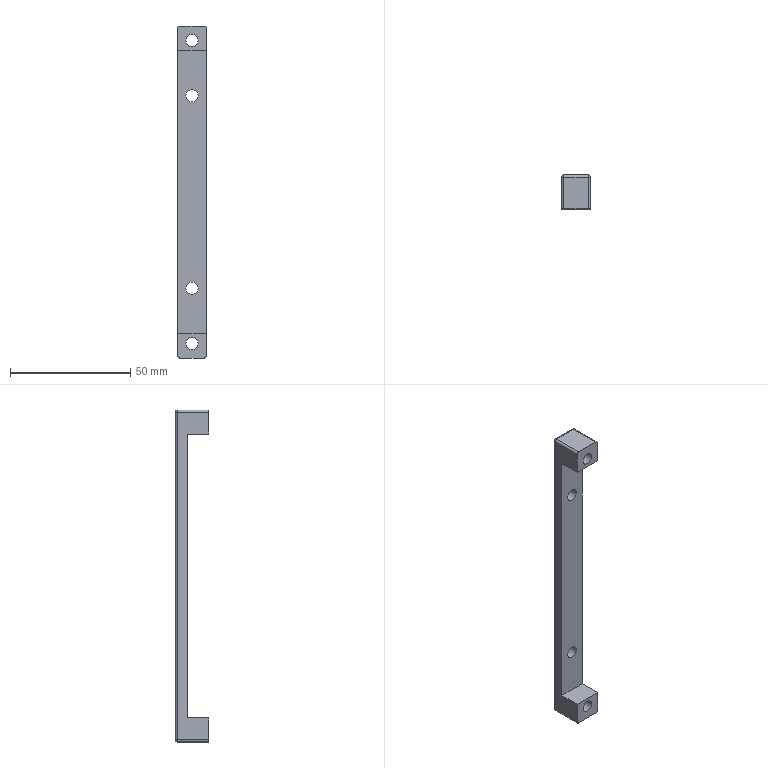Component | SolidWorks | 120.1-1 | 1 solid | 30 faces | box 12 x 14 x 138 mm | volume 9618 mm3 | cylinder 16 | plane 10 | sphere 4 | commonest cylinder face diameters 5 x8 2 x8
build123d program:
from build123d import *

# Parameters (mm, degrees)
SKETCH2_W                    = 138
SKETCH2_H                    = 12
BOSS_EXTRUDE1_DEPTH          = 14
SKETCH3_W                    = 118
SKETCH3_H                    = 9
CUT_EXTRUDE1_DEPTH           = 14
F_5_0_5_DIAMETER_HOLE1_D     = 5
F_5_0_5_DIAMETER_HOLE1_DEPTH = 15
F_5_0_5_DIAMETER_HOLE1_TIP   = 1.502
F_5_0_5_DIAMETER_HOLE2_D     = 5
F_5_0_5_DIAMETER_HOLE2_DEPTH = 10.1
F_5_0_5_DIAMETER_HOLE2_TIP   = 1.502
FILLET1_R                    = 1


with BuildPart() as part:
    # Sketch2 → Boss-Extrude1 (new body)
    with BuildSketch(Plane(origin=(0, 0, 0), x_dir=(1, 0, 0), z_dir=(0, 1, 0))):
        Rectangle(SKETCH2_W, SKETCH2_H)
    extrude(amount=BOSS_EXTRUDE1_DEPTH)

    # Sketch3 → Cut-Extrude1 (cut)
    with BuildSketch(Plane.XY.offset(6)):
        with Locations((0, 4.5)):
            Rectangle(SKETCH3_W, SKETCH3_H)
    extrude(amount=-CUT_EXTRUDE1_DEPTH, mode=Mode.SUBTRACT)

    # 5.0 _5_ Diameter Hole1
    with Locations(Plane.XZ):
        with Locations((-63, 0), (63, 0)):
            Hole(F_5_0_5_DIAMETER_HOLE1_D / 2, depth=F_5_0_5_DIAMETER_HOLE1_DEPTH)
            with Locations((0, 0, -(F_5_0_5_DIAMETER_HOLE1_DEPTH + F_5_0_5_DIAMETER_HOLE1_TIP / 2))):  # 118° drill point
                Cone(0, F_5_0_5_DIAMETER_HOLE1_D / 2, F_5_0_5_DIAMETER_HOLE1_TIP, mode=Mode.SUBTRACT)

    # 5.0 _5_ Diameter Hole2
    with Locations(Plane(origin=(0, 14, 0), x_dir=(-1, 0, 0), z_dir=(0, 1, 0))):
        with Locations((-40, 0), (40, 0)):
            Hole(F_5_0_5_DIAMETER_HOLE2_D / 2, depth=F_5_0_5_DIAMETER_HOLE2_DEPTH)
            with Locations((0, 0, -(F_5_0_5_DIAMETER_HOLE2_DEPTH + F_5_0_5_DIAMETER_HOLE2_TIP / 2))):  # 118° drill point
                Cone(0, F_5_0_5_DIAMETER_HOLE2_D / 2, F_5_0_5_DIAMETER_HOLE2_TIP, mode=Mode.SUBTRACT)

    # Fillet1
    fillet1_edges = [part.edges().sort_by_distance(p)[0] for p in [
        (69, 14, 0),
        (0, 14, -6),
        (-69, 14, 0),
        (0, 14, 6),
        (-69, 7, -6),
        (69, 7, -6),
        (69, 7, 6),
        (-69, 7, 6),
    ]]
    fillet(fillet1_edges, radius=FILLET1_R)


solid = part.part

# Placed as in the assembly
solid = solid.moved(Location((8, 150.5, 0), (0, 90, 0)))
STEP:
#1=CARTESIAN_POINT('',(0.2165,6.28,-1.575));
#2=VERTEX_POINT('',#1);
#3=CARTESIAN_POINT('',(0.4134,6.28,-1.575));
#4=VERTEX_POINT('',#3);
#5=CARTESIAN_POINT('',(0.315,6.28,-1.575));
#6=DIRECTION('',(-0.,1.,0.));
#7=DIRECTION('',(1.,0.,0.));
#8=AXIS2_PLACEMENT_3D('',#5,#6,#7);
#9=CIRCLE('',#8,0.09843);
#10=EDGE_CURVE('',#2,#4,#9,.T.);
#11=ORIENTED_EDGE('',*,*,#10,.F.);
#12=CARTESIAN_POINT('',(0.2165,6.476,-1.575));
#13=VERTEX_POINT('',#12);
#14=CARTESIAN_POINT('',(0.2165,6.476,-1.575));
#15=DIRECTION('',(-0.,1.,0.));
#16=VECTOR('',#15,39.37);
#17=LINE('',#14,#16);
#18=EDGE_CURVE('',#2,#13,#17,.T.);
#19=ORIENTED_EDGE('',*,*,#18,.T.);
#20=CARTESIAN_POINT('',(0.4134,6.476,-1.575));
#21=VERTEX_POINT('',#20);
#22=CARTESIAN_POINT('',(0.315,6.476,-1.575));
#23=DIRECTION('',(-0.,1.,0.));
#24=DIRECTION('',(1.,0.,0.));
#25=AXIS2_PLACEMENT_3D('',#22,#23,#24);
#26=CIRCLE('',#25,0.09843);
#27=EDGE_CURVE('',#13,#21,#26,.T.);
#28=ORIENTED_EDGE('',*,*,#27,.T.);
#29=CARTESIAN_POINT('',(0.4134,6.476,-1.575));
#30=DIRECTION('',(-0.,1.,0.));
#31=VECTOR('',#30,39.37);
#32=LINE('',#29,#31);
#33=EDGE_CURVE('',#4,#21,#32,.T.);
#34=ORIENTED_EDGE('',*,*,#33,.F.);
#35=EDGE_LOOP('',(#11,#19,#28,#34));
#36=FACE_OUTER_BOUND('',#35,.T.);
#37=CARTESIAN_POINT('',(0.315,6.476,-1.575));
#38=DIRECTION('',(-0.,1.,0.));
#39=DIRECTION('',(1.,0.,0.));
#40=AXIS2_PLACEMENT_3D('',#37,#38,#39);
#41=CYLINDRICAL_SURFACE('',#40,0.09843);
#42=ADVANCED_FACE('',(#36),#41,.F.);
#43=CARTESIAN_POINT('',(0.2165,6.28,1.575));
#44=VERTEX_POINT('',#43);
#45=CARTESIAN_POINT('',(0.4134,6.28,1.575));
#46=VERTEX_POINT('',#45);
#47=CARTESIAN_POINT('',(0.315,6.28,1.575));
#48=DIRECTION('',(-0.,1.,0.));
#49=DIRECTION('',(1.,0.,0.));
#50=AXIS2_PLACEMENT_3D('',#47,#48,#49);
#51=CIRCLE('',#50,0.09843);
#52=EDGE_CURVE('',#44,#46,#51,.T.);
#53=ORIENTED_EDGE('',*,*,#52,.F.);
#54=CARTESIAN_POINT('',(0.2165,6.476,1.575));
#55=VERTEX_POINT('',#54);
#56=CARTESIAN_POINT('',(0.2165,6.476,1.575));
#57=DIRECTION('',(-0.,1.,0.));
#58=VECTOR('',#57,39.37);
#59=LINE('',#56,#58);
#60=EDGE_CURVE('',#44,#55,#59,.T.);
#61=ORIENTED_EDGE('',*,*,#60,.T.);
#62=CARTESIAN_POINT('',(0.4134,6.476,1.575));
#63=VERTEX_POINT('',#62);
#64=CARTESIAN_POINT('',(0.315,6.476,1.575));
#65=DIRECTION('',(-0.,1.,0.));
#66=DIRECTION('',(1.,0.,0.));
#67=AXIS2_PLACEMENT_3D('',#64,#65,#66);
#68=CIRCLE('',#67,0.09843);
#69=EDGE_CURVE('',#55,#63,#68,.T.);
#70=ORIENTED_EDGE('',*,*,#69,.T.);
#71=CARTESIAN_POINT('',(0.4134,6.476,1.575));
#72=DIRECTION('',(-0.,1.,0.));
#73=VECTOR('',#72,39.37);
#74=LINE('',#71,#73);
#75=EDGE_CURVE('',#46,#63,#74,.T.);
#76=ORIENTED_EDGE('',*,*,#75,.F.);
#77=EDGE_LOOP('',(#53,#61,#70,#76));
#78=FACE_OUTER_BOUND('',#77,.T.);
#79=CARTESIAN_POINT('',(0.315,6.476,1.575));
#80=DIRECTION('',(-0.,1.,0.));
#81=DIRECTION('',(1.,0.,0.));
#82=AXIS2_PLACEMENT_3D('',#79,#80,#81);
#83=CYLINDRICAL_SURFACE('',#82,0.09843);
#84=ADVANCED_FACE('',(#78),#83,.F.);
#85=CARTESIAN_POINT('',(0.2165,6.476,2.48));
#86=VERTEX_POINT('',#85);
#87=CARTESIAN_POINT('',(0.4134,6.476,2.48));
#88=VERTEX_POINT('',#87);
#89=CARTESIAN_POINT('',(0.315,6.476,2.48));
#90=DIRECTION('',(-0.,1.,0.));
#91=DIRECTION('',(1.,0.,0.));
#92=AXIS2_PLACEMENT_3D('',#89,#90,#91);
#93=CIRCLE('',#92,0.09843);
#94=EDGE_CURVE('',#86,#88,#93,.T.);
#95=ORIENTED_EDGE('',*,*,#94,.T.);
#96=CARTESIAN_POINT('',(0.4134,5.925,2.48));
#97=VERTEX_POINT('',#96);
#98=CARTESIAN_POINT('',(0.4134,5.925,2.48));
#99=DIRECTION('',(0.,-1.,-0.));
#100=VECTOR('',#99,39.37);
#101=LINE('',#98,#100);
#102=EDGE_CURVE('',#88,#97,#101,.T.);
#103=ORIENTED_EDGE('',*,*,#102,.T.);
#104=CARTESIAN_POINT('',(0.2165,5.925,2.48));
#105=VERTEX_POINT('',#104);
#106=CARTESIAN_POINT('',(0.315,5.925,2.48));
#107=DIRECTION('',(0.,-1.,-0.));
#108=DIRECTION('',(-1.,0.,0.));
#109=AXIS2_PLACEMENT_3D('',#106,#107,#108);
#110=CIRCLE('',#109,0.09843);
#111=EDGE_CURVE('',#97,#105,#110,.T.);
#112=ORIENTED_EDGE('',*,*,#111,.T.);
#113=CARTESIAN_POINT('',(0.2165,5.925,2.48));
#114=DIRECTION('',(0.,-1.,-0.));
#115=VECTOR('',#114,39.37);
#116=LINE('',#113,#115);
#117=EDGE_CURVE('',#86,#105,#116,.T.);
#118=ORIENTED_EDGE('',*,*,#117,.F.);
#119=EDGE_LOOP('',(#95,#103,#112,#118));
#120=FACE_OUTER_BOUND('',#119,.T.);
#121=CARTESIAN_POINT('',(0.315,5.925,2.48));
#122=DIRECTION('',(0.,-1.,-0.));
#123=DIRECTION('',(-1.,0.,0.));
#124=AXIS2_PLACEMENT_3D('',#121,#122,#123);
#125=CYLINDRICAL_SURFACE('',#124,0.09843);
#126=ADVANCED_FACE('',(#120),#125,.F.);
#127=CARTESIAN_POINT('',(0.2165,6.476,-2.48));
#128=VERTEX_POINT('',#127);
#129=CARTESIAN_POINT('',(0.4134,6.476,-2.48));
#130=VERTEX_POINT('',#129);
#131=CARTESIAN_POINT('',(0.315,6.476,-2.48));
#132=DIRECTION('',(-0.,1.,0.));
#133=DIRECTION('',(1.,0.,0.));
#134=AXIS2_PLACEMENT_3D('',#131,#132,#133);
#135=CIRCLE('',#134,0.09843);
#136=EDGE_CURVE('',#128,#130,#135,.T.);
#137=ORIENTED_EDGE('',*,*,#136,.T.);
#138=CARTESIAN_POINT('',(0.4134,5.925,-2.48));
#139=VERTEX_POINT('',#138);
#140=CARTESIAN_POINT('',(0.4134,5.925,-2.48));
#141=DIRECTION('',(0.,-1.,-0.));
#142=VECTOR('',#141,39.37);
#143=LINE('',#140,#142);
#144=EDGE_CURVE('',#130,#139,#143,.T.);
#145=ORIENTED_EDGE('',*,*,#144,.T.);
#146=CARTESIAN_POINT('',(0.2165,5.925,-2.48));
#147=VERTEX_POINT('',#146);
#148=CARTESIAN_POINT('',(0.315,5.925,-2.48));
#149=DIRECTION('',(0.,-1.,-0.));
#150=DIRECTION('',(-1.,0.,0.));
#151=AXIS2_PLACEMENT_3D('',#148,#149,#150);
#152=CIRCLE('',#151,0.09843);
#153=EDGE_CURVE('',#139,#147,#152,.T.);
#154=ORIENTED_EDGE('',*,*,#153,.T.);
#155=CARTESIAN_POINT('',(0.2165,5.925,-2.48));
#156=DIRECTION('',(0.,-1.,-0.));
#157=VECTOR('',#156,39.37);
#158=LINE('',#155,#157);
#159=EDGE_CURVE('',#128,#147,#158,.T.);
#160=ORIENTED_EDGE('',*,*,#159,.F.);
#161=EDGE_LOOP('',(#137,#145,#154,#160));
#162=FACE_OUTER_BOUND('',#161,.T.);
#163=CARTESIAN_POINT('',(0.315,5.925,-2.48));
#164=DIRECTION('',(0.,-1.,-0.));
#165=DIRECTION('',(-1.,0.,0.));
#166=AXIS2_PLACEMENT_3D('',#163,#164,#165);
#167=CYLINDRICAL_SURFACE('',#166,0.09843);
#168=ADVANCED_FACE('',(#162),#167,.F.);
#169=CARTESIAN_POINT('',(0.315,5.925,2.48));
#170=DIRECTION('',(0.,-1.,-0.));
#171=DIRECTION('',(-1.,0.,0.));
#172=AXIS2_PLACEMENT_3D('',#169,#170,#171);
#173=CIRCLE('',#172,0.09843);
#174=EDGE_CURVE('',#105,#97,#173,.T.);
#175=ORIENTED_EDGE('',*,*,#174,.F.);
#176=ORIENTED_EDGE('',*,*,#111,.F.);
#177=EDGE_LOOP('',(#175,#176));
#178=FACE_BOUND('',#177,.T.);
#179=CARTESIAN_POINT('',(0.1181,5.925,2.717));
#180=VERTEX_POINT('',#179);
#181=CARTESIAN_POINT('',(0.5118,5.925,2.717));
#182=VERTEX_POINT('',#181);
#183=CARTESIAN_POINT('',(0.5512,5.925,2.717));
#184=DIRECTION('',(1.,0.,-0.));
#185=VECTOR('',#184,39.37);
#186=LINE('',#183,#185);
#187=EDGE_CURVE('',#180,#182,#186,.T.);
#188=ORIENTED_EDGE('',*,*,#187,.F.);
#189=CARTESIAN_POINT('',(0.07874,5.925,2.677));
#190=VERTEX_POINT('',#189);
#191=CARTESIAN_POINT('',(0.1181,5.925,2.677));
#192=DIRECTION('',(0.,-1.,-0.));
#193=DIRECTION('',(1.,0.,0.));
#194=AXIS2_PLACEMENT_3D('',#191,#192,#193);
#195=CIRCLE('',#194,0.03937);
#196=EDGE_CURVE('',#180,#190,#195,.T.);
#197=ORIENTED_EDGE('',*,*,#196,.T.);
#198=CARTESIAN_POINT('',(0.07874,5.925,2.323));
#199=VERTEX_POINT('',#198);
#200=CARTESIAN_POINT('',(0.07874,5.925,-2.717));
#201=DIRECTION('',(0.,-0.,1.));
#202=VECTOR('',#201,39.37);
#203=LINE('',#200,#202);
#204=EDGE_CURVE('',#199,#190,#203,.T.);
#205=ORIENTED_EDGE('',*,*,#204,.F.);
#206=CARTESIAN_POINT('',(0.5512,5.925,2.323));
#207=VERTEX_POINT('',#206);
#208=CARTESIAN_POINT('',(0.07874,5.925,2.323));
#209=DIRECTION('',(1.,0.,-0.));
#210=VECTOR('',#209,39.37);
#211=LINE('',#208,#210);
#212=EDGE_CURVE('',#199,#207,#211,.T.);
#213=ORIENTED_EDGE('',*,*,#212,.T.);
#214=CARTESIAN_POINT('',(0.5512,5.925,2.677));
#215=VERTEX_POINT('',#214);
#216=CARTESIAN_POINT('',(0.5512,5.925,-2.717));
#217=DIRECTION('',(-0.,0.,-1.));
#218=VECTOR('',#217,39.37);
#219=LINE('',#216,#218);
#220=EDGE_CURVE('',#215,#207,#219,.T.);
#221=ORIENTED_EDGE('',*,*,#220,.F.);
#222=CARTESIAN_POINT('',(0.5118,5.925,2.677));
#223=DIRECTION('',(0.,-1.,-0.));
#224=DIRECTION('',(1.,0.,0.));
#225=AXIS2_PLACEMENT_3D('',#222,#223,#224);
#226=CIRCLE('',#225,0.03937);
#227=EDGE_CURVE('',#215,#182,#226,.T.);
#228=ORIENTED_EDGE('',*,*,#227,.T.);
#229=EDGE_LOOP('',(#188,#197,#205,#213,#221,#228));
#230=FACE_OUTER_BOUND('',#229,.T.);
#231=CARTESIAN_POINT('',(0.07874,5.925,2.717));
#232=DIRECTION('',(-0.,1.,0.));
#233=DIRECTION('',(1.,0.,-0.));
#234=AXIS2_PLACEMENT_3D('',#231,#232,#233);
#235=PLANE('',#234);
#236=ADVANCED_FACE('',(#178,#230),#235,.F.);
#237=CARTESIAN_POINT('',(0.5118,6.437,2.717));
#238=VERTEX_POINT('',#237);
#239=CARTESIAN_POINT('',(0.1181,6.437,2.717));
#240=VERTEX_POINT('',#239);
#241=CARTESIAN_POINT('',(0.07874,6.437,2.717));
#242=DIRECTION('',(-1.,-0.,0.));
#243=VECTOR('',#242,39.37);
#244=LINE('',#241,#243);
#245=EDGE_CURVE('',#238,#240,#244,.T.);
#246=ORIENTED_EDGE('',*,*,#245,.T.);
#247=CARTESIAN_POINT('',(0.1181,6.476,2.717));
#248=DIRECTION('',(0.,-1.,-0.));
#249=VECTOR('',#248,39.37);
#250=LINE('',#247,#249);
#251=EDGE_CURVE('',#240,#180,#250,.T.);
#252=ORIENTED_EDGE('',*,*,#251,.T.);
#253=ORIENTED_EDGE('',*,*,#187,.T.);
#254=CARTESIAN_POINT('',(0.5118,6.476,2.717));
#255=DIRECTION('',(-0.,1.,0.));
#256=VECTOR('',#255,39.37);
#257=LINE('',#254,#256);
#258=EDGE_CURVE('',#182,#238,#257,.T.);
#259=ORIENTED_EDGE('',*,*,#258,.T.);
#260=EDGE_LOOP('',(#246,#252,#253,#259));
#261=FACE_OUTER_BOUND('',#260,.T.);
#262=CARTESIAN_POINT('',(0.5512,6.476,2.717));
#263=DIRECTION('',(-0.,0.,-1.));
#264=DIRECTION('',(-1.,-0.,0.));
#265=AXIS2_PLACEMENT_3D('',#262,#263,#264);
#266=PLANE('',#265);
#267=ADVANCED_FACE('',(#261),#266,.F.);
#268=CARTESIAN_POINT('',(0.5512,5.925,-2.323));
#269=VERTEX_POINT('',#268);
#270=CARTESIAN_POINT('',(0.5512,5.925,-2.677));
#271=VERTEX_POINT('',#270);
#272=CARTESIAN_POINT('',(0.5512,5.925,-2.717));
#273=DIRECTION('',(-0.,0.,-1.));
#274=VECTOR('',#273,39.37);
#275=LINE('',#272,#274);
#276=EDGE_CURVE('',#269,#271,#275,.T.);
#277=ORIENTED_EDGE('',*,*,#276,.T.);
#278=CARTESIAN_POINT('',(0.5512,6.437,-2.677));
#279=VERTEX_POINT('',#278);
#280=CARTESIAN_POINT('',(0.5512,6.476,-2.677));
#281=DIRECTION('',(-0.,1.,0.));
#282=VECTOR('',#281,39.37);
#283=LINE('',#280,#282);
#284=EDGE_CURVE('',#271,#279,#283,.T.);
#285=ORIENTED_EDGE('',*,*,#284,.T.);
#286=CARTESIAN_POINT('',(0.5512,6.437,2.677));
#287=VERTEX_POINT('',#286);
#288=CARTESIAN_POINT('',(0.5512,6.437,2.717));
#289=DIRECTION('',(0.,-0.,1.));
#290=VECTOR('',#289,39.37);
#291=LINE('',#288,#290);
#292=EDGE_CURVE('',#279,#287,#291,.T.);
#293=ORIENTED_EDGE('',*,*,#292,.T.);
#294=CARTESIAN_POINT('',(0.5512,6.476,2.677));
#295=DIRECTION('',(0.,-1.,-0.));
#296=VECTOR('',#295,39.37);
#297=LINE('',#294,#296);
#298=EDGE_CURVE('',#287,#215,#297,.T.);
#299=ORIENTED_EDGE('',*,*,#298,.T.);
#300=ORIENTED_EDGE('',*,*,#220,.T.);
#301=CARTESIAN_POINT('',(0.5512,6.28,2.323));
#302=VERTEX_POINT('',#301);
#303=CARTESIAN_POINT('',(0.5512,5.925,2.323));
#304=DIRECTION('',(0.,-1.,-0.));
#305=VECTOR('',#304,39.37);
#306=LINE('',#303,#305);
#307=EDGE_CURVE('',#302,#207,#306,.T.);
#308=ORIENTED_EDGE('',*,*,#307,.F.);
#309=CARTESIAN_POINT('',(0.5512,6.28,-2.323));
#310=VERTEX_POINT('',#309);
#311=CARTESIAN_POINT('',(0.5512,6.28,2.323));
#312=DIRECTION('',(0.,-0.,1.));
#313=VECTOR('',#312,39.37);
#314=LINE('',#311,#313);
#315=EDGE_CURVE('',#310,#302,#314,.T.);
#316=ORIENTED_EDGE('',*,*,#315,.F.);
#317=CARTESIAN_POINT('',(0.5512,5.925,-2.323));
#318=DIRECTION('',(-0.,1.,0.));
#319=VECTOR('',#318,39.37);
#320=LINE('',#317,#319);
#321=EDGE_CURVE('',#269,#310,#320,.T.);
#322=ORIENTED_EDGE('',*,*,#321,.F.);
#323=EDGE_LOOP('',(#277,#285,#293,#299,#300,#308,#316,#322));
#324=FACE_OUTER_BOUND('',#323,.T.);
#325=CARTESIAN_POINT('',(0.5512,6.476,-2.717));
#326=DIRECTION('',(-1.,-0.,0.));
#327=DIRECTION('',(0.,-0.,1.));
#328=AXIS2_PLACEMENT_3D('',#325,#326,#327);
#329=PLANE('',#328);
#330=ADVANCED_FACE('',(#324),#329,.F.);
#331=CARTESIAN_POINT('',(0.5118,5.925,-2.717));
#332=VERTEX_POINT('',#331);
#333=CARTESIAN_POINT('',(0.1181,5.925,-2.717));
#334=VERTEX_POINT('',#333);
#335=CARTESIAN_POINT('',(0.5512,5.925,-2.717));
#336=DIRECTION('',(-1.,-0.,0.));
#337=VECTOR('',#336,39.37);
#338=LINE('',#335,#337);
#339=EDGE_CURVE('',#332,#334,#338,.T.);
#340=ORIENTED_EDGE('',*,*,#339,.T.);
#341=CARTESIAN_POINT('',(0.1181,6.437,-2.717));
#342=VERTEX_POINT('',#341);
#343=CARTESIAN_POINT('',(0.1181,6.476,-2.717));
#344=DIRECTION('',(-0.,1.,0.));
#345=VECTOR('',#344,39.37);
#346=LINE('',#343,#345);
#347=EDGE_CURVE('',#334,#342,#346,.T.);
#348=ORIENTED_EDGE('',*,*,#347,.T.);
#349=CARTESIAN_POINT('',(0.5118,6.437,-2.717));
#350=VERTEX_POINT('',#349);
#351=CARTESIAN_POINT('',(0.5512,6.437,-2.717));
#352=DIRECTION('',(1.,0.,-0.));
#353=VECTOR('',#352,39.37);
#354=LINE('',#351,#353);
#355=EDGE_CURVE('',#342,#350,#354,.T.);
#356=ORIENTED_EDGE('',*,*,#355,.T.);
#357=CARTESIAN_POINT('',(0.5118,6.476,-2.717));
#358=DIRECTION('',(0.,-1.,-0.));
#359=VECTOR('',#358,39.37);
#360=LINE('',#357,#359);
#361=EDGE_CURVE('',#350,#332,#360,.T.);
#362=ORIENTED_EDGE('',*,*,#361,.T.);
#363=EDGE_LOOP('',(#340,#348,#356,#362));
#364=FACE_OUTER_BOUND('',#363,.T.);
#365=CARTESIAN_POINT('',(0.5512,6.476,-2.717));
#366=DIRECTION('',(0.,-0.,1.));
#367=DIRECTION('',(1.,0.,-0.));
#368=AXIS2_PLACEMENT_3D('',#365,#366,#367);
#369=PLANE('',#368);
#370=ADVANCED_FACE('',(#364),#369,.F.);
#371=CARTESIAN_POINT('',(0.07874,6.437,2.677));
#372=VERTEX_POINT('',#371);
#373=CARTESIAN_POINT('',(0.07874,6.437,-2.677));
#374=VERTEX_POINT('',#373);
#375=CARTESIAN_POINT('',(0.07874,6.437,-2.717));
#376=DIRECTION('',(-0.,0.,-1.));
#377=VECTOR('',#376,39.37);
#378=LINE('',#375,#377);
#379=EDGE_CURVE('',#372,#374,#378,.T.);
#380=ORIENTED_EDGE('',*,*,#379,.T.);
#381=CARTESIAN_POINT('',(0.07874,5.925,-2.677));
#382=VERTEX_POINT('',#381);
#383=CARTESIAN_POINT('',(0.07874,6.476,-2.677));
#384=DIRECTION('',(0.,-1.,-0.));
#385=VECTOR('',#384,39.37);
#386=LINE('',#383,#385);
#387=EDGE_CURVE('',#374,#382,#386,.T.);
#388=ORIENTED_EDGE('',*,*,#387,.T.);
#389=CARTESIAN_POINT('',(0.07874,5.925,-2.323));
#390=VERTEX_POINT('',#389);
#391=CARTESIAN_POINT('',(0.07874,5.925,-2.717));
#392=DIRECTION('',(0.,-0.,1.));
#393=VECTOR('',#392,39.37);
#394=LINE('',#391,#393);
#395=EDGE_CURVE('',#382,#390,#394,.T.);
#396=ORIENTED_EDGE('',*,*,#395,.T.);
#397=CARTESIAN_POINT('',(0.07874,6.28,-2.323));
#398=VERTEX_POINT('',#397);
#399=CARTESIAN_POINT('',(0.07874,6.476,-2.323));
#400=DIRECTION('',(-0.,1.,0.));
#401=VECTOR('',#400,39.37);
#402=LINE('',#399,#401);
#403=EDGE_CURVE('',#390,#398,#402,.T.);
#404=ORIENTED_EDGE('',*,*,#403,.T.);
#405=CARTESIAN_POINT('',(0.07874,6.28,2.323));
#406=VERTEX_POINT('',#405);
#407=CARTESIAN_POINT('',(0.07874,6.28,-2.717));
#408=DIRECTION('',(0.,-0.,1.));
#409=VECTOR('',#408,39.37);
#410=LINE('',#407,#409);
#411=EDGE_CURVE('',#398,#406,#410,.T.);
#412=ORIENTED_EDGE('',*,*,#411,.T.);
#413=CARTESIAN_POINT('',(0.07874,6.476,2.323));
#414=DIRECTION('',(0.,-1.,-0.));
#415=VECTOR('',#414,39.37);
#416=LINE('',#413,#415);
#417=EDGE_CURVE('',#406,#199,#416,.T.);
#418=ORIENTED_EDGE('',*,*,#417,.T.);
#419=ORIENTED_EDGE('',*,*,#204,.T.);
#420=CARTESIAN_POINT('',(0.07874,6.476,2.677));
#421=DIRECTION('',(-0.,1.,0.));
#422=VECTOR('',#421,39.37);
#423=LINE('',#420,#422);
#424=EDGE_CURVE('',#190,#372,#423,.T.);
#425=ORIENTED_EDGE('',*,*,#424,.T.);
#426=EDGE_LOOP('',(#380,#388,#396,#404,#412,#418,#419,#425));
#427=FACE_OUTER_BOUND('',#426,.T.);
#428=CARTESIAN_POINT('',(0.07874,6.476,-2.717));
#429=DIRECTION('',(1.,0.,-0.));
#430=DIRECTION('',(-0.,0.,-1.));
#431=AXIS2_PLACEMENT_3D('',#428,#429,#430);
#432=PLANE('',#431);
#433=ADVANCED_FACE('',(#427),#432,.F.);
#434=CARTESIAN_POINT('',(0.5118,6.476,-2.677));
#435=VERTEX_POINT('',#434);
#436=CARTESIAN_POINT('',(0.1181,6.476,-2.677));
#437=VERTEX_POINT('',#436);
#438=CARTESIAN_POINT('',(0.07874,6.476,-2.677));
#439=DIRECTION('',(-1.,-0.,0.));
#440=VECTOR('',#439,39.37);
#441=LINE('',#438,#440);
#442=EDGE_CURVE('',#435,#437,#441,.T.);
#443=ORIENTED_EDGE('',*,*,#442,.T.);
#444=CARTESIAN_POINT('',(0.1181,6.476,2.677));
#445=VERTEX_POINT('',#444);
#446=CARTESIAN_POINT('',(0.1181,6.476,2.717));
#447=DIRECTION('',(0.,-0.,1.));
#448=VECTOR('',#447,39.37);
#449=LINE('',#446,#448);
#450=EDGE_CURVE('',#437,#445,#449,.T.);
#451=ORIENTED_EDGE('',*,*,#450,.T.);
#452=CARTESIAN_POINT('',(0.5118,6.476,2.677));
#453=VERTEX_POINT('',#452);
#454=CARTESIAN_POINT('',(0.5512,6.476,2.677));
#455=DIRECTION('',(1.,0.,-0.));
#456=VECTOR('',#455,39.37);
#457=LINE('',#454,#456);
#458=EDGE_CURVE('',#445,#453,#457,.T.);
#459=ORIENTED_EDGE('',*,*,#458,.T.);
#460=CARTESIAN_POINT('',(0.5118,6.476,-2.717));
#461=DIRECTION('',(-0.,0.,-1.));
#462=VECTOR('',#461,39.37);
#463=LINE('',#460,#462);
#464=EDGE_CURVE('',#453,#435,#463,.T.);
#465=ORIENTED_EDGE('',*,*,#464,.T.);
#466=EDGE_LOOP('',(#443,#451,#459,#465));
#467=FACE_OUTER_BOUND('',#466,.T.);
#468=CARTESIAN_POINT('',(0.315,6.476,-1.575));
#469=DIRECTION('',(-0.,1.,0.));
#470=DIRECTION('',(1.,0.,0.));
#471=AXIS2_PLACEMENT_3D('',#468,#469,#470);
#472=CIRCLE('',#471,0.09843);
#473=EDGE_CURVE('',#21,#13,#472,.T.);
#474=ORIENTED_EDGE('',*,*,#473,.F.);
#475=ORIENTED_EDGE('',*,*,#27,.F.);
#476=EDGE_LOOP('',(#474,#475));
#477=FACE_BOUND('',#476,.T.);
#478=CARTESIAN_POINT('',(0.315,6.476,1.575));
#479=DIRECTION('',(-0.,1.,0.));
#480=DIRECTION('',(1.,0.,0.));
#481=AXIS2_PLACEMENT_3D('',#478,#479,#480);
#482=CIRCLE('',#481,0.09843);
#483=EDGE_CURVE('',#63,#55,#482,.T.);
#484=ORIENTED_EDGE('',*,*,#483,.F.);
#485=ORIENTED_EDGE('',*,*,#69,.F.);
#486=EDGE_LOOP('',(#484,#485));
#487=FACE_BOUND('',#486,.T.);
#488=ORIENTED_EDGE('',*,*,#94,.F.);
#489=CARTESIAN_POINT('',(0.315,6.476,2.48));
#490=DIRECTION('',(-0.,1.,0.));
#491=DIRECTION('',(1.,0.,0.));
#492=AXIS2_PLACEMENT_3D('',#489,#490,#491);
#493=CIRCLE('',#492,0.09843);
#494=EDGE_CURVE('',#88,#86,#493,.T.);
#495=ORIENTED_EDGE('',*,*,#494,.F.);
#496=EDGE_LOOP('',(#488,#495));
#497=FACE_BOUND('',#496,.T.);
#498=ORIENTED_EDGE('',*,*,#136,.F.);
#499=CARTESIAN_POINT('',(0.315,6.476,-2.48));
#500=DIRECTION('',(-0.,1.,0.));
#501=DIRECTION('',(1.,0.,0.));
#502=AXIS2_PLACEMENT_3D('',#499,#500,#501);
#503=CIRCLE('',#502,0.09843);
#504=EDGE_CURVE('',#130,#128,#503,.T.);
#505=ORIENTED_EDGE('',*,*,#504,.F.);
#506=EDGE_LOOP('',(#498,#505));
#507=FACE_BOUND('',#506,.T.);
#508=CARTESIAN_POINT('',(0.07874,6.476,2.717));
#509=DIRECTION('',(-0.,1.,0.));
#510=DIRECTION('',(1.,0.,-0.));
#511=AXIS2_PLACEMENT_3D('',#508,#509,#510);
#512=PLANE('',#511);
#513=ADVANCED_FACE('',(#467,#477,#487,#497,#507),#512,.T.);
#514=CARTESIAN_POINT('',(0.315,5.925,-2.48));
#515=DIRECTION('',(0.,-1.,-0.));
#516=DIRECTION('',(-1.,0.,0.));
#517=AXIS2_PLACEMENT_3D('',#514,#515,#516);
#518=CIRCLE('',#517,0.09843);
#519=EDGE_CURVE('',#147,#139,#518,.T.);
#520=ORIENTED_EDGE('',*,*,#519,.F.);
#521=ORIENTED_EDGE('',*,*,#153,.F.);
#522=EDGE_LOOP('',(#520,#521));
#523=FACE_BOUND('',#522,.T.);
#524=ORIENTED_EDGE('',*,*,#395,.F.);
#525=CARTESIAN_POINT('',(0.1181,5.925,-2.677));
#526=DIRECTION('',(0.,-1.,-0.));
#527=DIRECTION('',(1.,0.,0.));
#528=AXIS2_PLACEMENT_3D('',#525,#526,#527);
#529=CIRCLE('',#528,0.03937);
#530=EDGE_CURVE('',#382,#334,#529,.T.);
#531=ORIENTED_EDGE('',*,*,#530,.T.);
#532=ORIENTED_EDGE('',*,*,#339,.F.);
#533=CARTESIAN_POINT('',(0.5118,5.925,-2.677));
#534=DIRECTION('',(0.,-1.,-0.));
#535=DIRECTION('',(1.,0.,0.));
#536=AXIS2_PLACEMENT_3D('',#533,#534,#535);
#537=CIRCLE('',#536,0.03937);
#538=EDGE_CURVE('',#332,#271,#537,.T.);
#539=ORIENTED_EDGE('',*,*,#538,.T.);
#540=ORIENTED_EDGE('',*,*,#276,.F.);
#541=CARTESIAN_POINT('',(0.07874,5.925,-2.323));
#542=DIRECTION('',(-1.,-0.,0.));
#543=VECTOR('',#542,39.37);
#544=LINE('',#541,#543);
#545=EDGE_CURVE('',#269,#390,#544,.T.);
#546=ORIENTED_EDGE('',*,*,#545,.T.);
#547=EDGE_LOOP('',(#524,#531,#532,#539,#540,#546));
#548=FACE_OUTER_BOUND('',#547,.T.);
#549=CARTESIAN_POINT('',(0.07874,5.925,2.717));
#550=DIRECTION('',(-0.,1.,0.));
#551=DIRECTION('',(1.,0.,-0.));
#552=AXIS2_PLACEMENT_3D('',#549,#550,#551);
#553=PLANE('',#552);
#554=ADVANCED_FACE('',(#523,#548),#553,.F.);
#555=CARTESIAN_POINT('',(0.315,6.28,-1.575));
#556=DIRECTION('',(-0.,1.,0.));
#557=DIRECTION('',(1.,0.,0.));
#558=AXIS2_PLACEMENT_3D('',#555,#556,#557);
#559=CIRCLE('',#558,0.09843);
#560=EDGE_CURVE('',#4,#2,#559,.T.);
#561=ORIENTED_EDGE('',*,*,#560,.T.);
#562=ORIENTED_EDGE('',*,*,#10,.T.);
#563=EDGE_LOOP('',(#561,#562));
#564=FACE_BOUND('',#563,.T.);
#565=CARTESIAN_POINT('',(0.315,6.28,1.575));
#566=DIRECTION('',(-0.,1.,0.));
#567=DIRECTION('',(1.,0.,0.));
#568=AXIS2_PLACEMENT_3D('',#565,#566,#567);
#569=CIRCLE('',#568,0.09843);
#570=EDGE_CURVE('',#46,#44,#569,.T.);
#571=ORIENTED_EDGE('',*,*,#570,.T.);
#572=ORIENTED_EDGE('',*,*,#52,.T.);
#573=EDGE_LOOP('',(#571,#572));
#574=FACE_BOUND('',#573,.T.);
#575=CARTESIAN_POINT('',(0.,6.28,-2.323));
#576=DIRECTION('',(1.,0.,-0.));
#577=VECTOR('',#576,39.37);
#578=LINE('',#575,#577);
#579=EDGE_CURVE('',#398,#310,#578,.T.);
#580=ORIENTED_EDGE('',*,*,#579,.T.);
#581=ORIENTED_EDGE('',*,*,#315,.T.);
#582=CARTESIAN_POINT('',(0.,6.28,2.323));
#583=DIRECTION('',(1.,0.,-0.));
#584=VECTOR('',#583,39.37);
#585=LINE('',#582,#584);
#586=EDGE_CURVE('',#406,#302,#585,.T.);
#587=ORIENTED_EDGE('',*,*,#586,.F.);
#588=ORIENTED_EDGE('',*,*,#411,.F.);
#589=EDGE_LOOP('',(#580,#581,#587,#588));
#590=FACE_OUTER_BOUND('',#589,.T.);
#591=CARTESIAN_POINT('',(0.,6.28,2.323));
#592=DIRECTION('',(-0.,1.,0.));
#593=DIRECTION('',(1.,0.,-0.));
#594=AXIS2_PLACEMENT_3D('',#591,#592,#593);
#595=PLANE('',#594);
#596=ADVANCED_FACE('',(#564,#574,#590),#595,.F.);
#597=ORIENTED_EDGE('',*,*,#586,.T.);
#598=ORIENTED_EDGE('',*,*,#307,.T.);
#599=ORIENTED_EDGE('',*,*,#212,.F.);
#600=ORIENTED_EDGE('',*,*,#417,.F.);
#601=EDGE_LOOP('',(#597,#598,#599,#600));
#602=FACE_OUTER_BOUND('',#601,.T.);
#603=CARTESIAN_POINT('',(0.,5.925,2.323));
#604=DIRECTION('',(0.,-0.,1.));
#605=DIRECTION('',(1.,0.,-0.));
#606=AXIS2_PLACEMENT_3D('',#603,#604,#605);
#607=PLANE('',#606);
#608=ADVANCED_FACE('',(#602),#607,.F.);
#609=ORIENTED_EDGE('',*,*,#545,.F.);
#610=ORIENTED_EDGE('',*,*,#321,.T.);
#611=ORIENTED_EDGE('',*,*,#579,.F.);
#612=ORIENTED_EDGE('',*,*,#403,.F.);
#613=EDGE_LOOP('',(#609,#610,#611,#612));
#614=FACE_OUTER_BOUND('',#613,.T.);
#615=CARTESIAN_POINT('',(0.,5.925,-2.323));
#616=DIRECTION('',(-0.,0.,-1.));
#617=DIRECTION('',(-1.,-0.,0.));
#618=AXIS2_PLACEMENT_3D('',#615,#616,#617);
#619=PLANE('',#618);
#620=ADVANCED_FACE('',(#614),#619,.F.);
#621=ORIENTED_EDGE('',*,*,#144,.F.);
#622=ORIENTED_EDGE('',*,*,#504,.T.);
#623=ORIENTED_EDGE('',*,*,#159,.T.);
#624=ORIENTED_EDGE('',*,*,#519,.T.);
#625=EDGE_LOOP('',(#621,#622,#623,#624));
#626=FACE_OUTER_BOUND('',#625,.T.);
#627=CARTESIAN_POINT('',(0.315,5.925,-2.48));
#628=DIRECTION('',(0.,-1.,-0.));
#629=DIRECTION('',(-1.,0.,0.));
#630=AXIS2_PLACEMENT_3D('',#627,#628,#629);
#631=CYLINDRICAL_SURFACE('',#630,0.09843);
#632=ADVANCED_FACE('',(#626),#631,.F.);
#633=ORIENTED_EDGE('',*,*,#102,.F.);
#634=ORIENTED_EDGE('',*,*,#494,.T.);
#635=ORIENTED_EDGE('',*,*,#117,.T.);
#636=ORIENTED_EDGE('',*,*,#174,.T.);
#637=EDGE_LOOP('',(#633,#634,#635,#636));
#638=FACE_OUTER_BOUND('',#637,.T.);
#639=CARTESIAN_POINT('',(0.315,5.925,2.48));
#640=DIRECTION('',(0.,-1.,-0.));
#641=DIRECTION('',(-1.,0.,0.));
#642=AXIS2_PLACEMENT_3D('',#639,#640,#641);
#643=CYLINDRICAL_SURFACE('',#642,0.09843);
#644=ADVANCED_FACE('',(#638),#643,.F.);
#645=ORIENTED_EDGE('',*,*,#60,.F.);
#646=ORIENTED_EDGE('',*,*,#570,.F.);
#647=ORIENTED_EDGE('',*,*,#75,.T.);
#648=ORIENTED_EDGE('',*,*,#483,.T.);
#649=EDGE_LOOP('',(#645,#646,#647,#648));
#650=FACE_OUTER_BOUND('',#649,.T.);
#651=CARTESIAN_POINT('',(0.315,6.476,1.575));
#652=DIRECTION('',(-0.,1.,0.));
#653=DIRECTION('',(1.,0.,0.));
#654=AXIS2_PLACEMENT_3D('',#651,#652,#653);
#655=CYLINDRICAL_SURFACE('',#654,0.09843);
#656=ADVANCED_FACE('',(#650),#655,.F.);
#657=ORIENTED_EDGE('',*,*,#18,.F.);
#658=ORIENTED_EDGE('',*,*,#560,.F.);
#659=ORIENTED_EDGE('',*,*,#33,.T.);
#660=ORIENTED_EDGE('',*,*,#473,.T.);
#661=EDGE_LOOP('',(#657,#658,#659,#660));
#662=FACE_OUTER_BOUND('',#661,.T.);
#663=CARTESIAN_POINT('',(0.315,6.476,-1.575));
#664=DIRECTION('',(-0.,1.,0.));
#665=DIRECTION('',(1.,0.,0.));
#666=AXIS2_PLACEMENT_3D('',#663,#664,#665);
#667=CYLINDRICAL_SURFACE('',#666,0.09843);
#668=ADVANCED_FACE('',(#662),#667,.F.);
#669=CARTESIAN_POINT('',(0.5118,6.437,2.677));
#670=DIRECTION('',(-0.,1.,0.));
#671=DIRECTION('',(1.,0.,0.));
#672=AXIS2_PLACEMENT_3D('',#669,#670,#671);
#673=CIRCLE('',#672,0.03937);
#674=EDGE_CURVE('',#238,#287,#673,.T.);
#675=ORIENTED_EDGE('',*,*,#674,.F.);
#676=ORIENTED_EDGE('',*,*,#258,.F.);
#677=ORIENTED_EDGE('',*,*,#227,.F.);
#678=ORIENTED_EDGE('',*,*,#298,.F.);
#679=EDGE_LOOP('',(#675,#676,#677,#678));
#680=FACE_OUTER_BOUND('',#679,.T.);
#681=CARTESIAN_POINT('',(0.5118,6.476,2.677));
#682=DIRECTION('',(0.,-1.,-0.));
#683=DIRECTION('',(-1.,0.,0.));
#684=AXIS2_PLACEMENT_3D('',#681,#682,#683);
#685=CYLINDRICAL_SURFACE('',#684,0.03937);
#686=ADVANCED_FACE('',(#680),#685,.T.);
#687=CARTESIAN_POINT('',(0.5118,6.437,2.677));
#688=DIRECTION('',(-1.,-0.,0.));
#689=DIRECTION('',(-0.,0.,-1.));
#690=AXIS2_PLACEMENT_3D('',#687,#688,#689);
#691=CIRCLE('',#690,0.03937);
#692=EDGE_CURVE('',#238,#453,#691,.T.);
#693=ORIENTED_EDGE('',*,*,#692,.F.);
#694=ORIENTED_EDGE('',*,*,#674,.T.);
#695=CARTESIAN_POINT('',(0.5118,6.437,2.677));
#696=DIRECTION('',(-0.,0.,-1.));
#697=DIRECTION('',(1.,0.,0.));
#698=AXIS2_PLACEMENT_3D('',#695,#696,#697);
#699=CIRCLE('',#698,0.03937);
#700=EDGE_CURVE('',#453,#287,#699,.T.);
#701=ORIENTED_EDGE('',*,*,#700,.F.);
#702=EDGE_LOOP('',(#693,#694,#701));
#703=FACE_OUTER_BOUND('',#702,.T.);
#704=CARTESIAN_POINT('',(0.5118,6.437,2.677));
#705=DIRECTION('',(-0.,1.,0.));
#706=DIRECTION('',(0.,0.,-1.));
#707=AXIS2_PLACEMENT_3D('',#704,#705,#706);
#708=SPHERICAL_SURFACE('',#707,0.03937);
#709=ADVANCED_FACE('',(#703),#708,.T.);
#710=ORIENTED_EDGE('',*,*,#538,.F.);
#711=ORIENTED_EDGE('',*,*,#361,.F.);
#712=CARTESIAN_POINT('',(0.5118,6.437,-2.677));
#713=DIRECTION('',(-0.,1.,0.));
#714=DIRECTION('',(1.,0.,0.));
#715=AXIS2_PLACEMENT_3D('',#712,#713,#714);
#716=CIRCLE('',#715,0.03937);
#717=EDGE_CURVE('',#279,#350,#716,.T.);
#718=ORIENTED_EDGE('',*,*,#717,.F.);
#719=ORIENTED_EDGE('',*,*,#284,.F.);
#720=EDGE_LOOP('',(#710,#711,#718,#719));
#721=FACE_OUTER_BOUND('',#720,.T.);
#722=CARTESIAN_POINT('',(0.5118,6.476,-2.677));
#723=DIRECTION('',(0.,-1.,-0.));
#724=DIRECTION('',(-1.,0.,0.));
#725=AXIS2_PLACEMENT_3D('',#722,#723,#724);
#726=CYLINDRICAL_SURFACE('',#725,0.03937);
#727=ADVANCED_FACE('',(#721),#726,.T.);
#728=ORIENTED_EDGE('',*,*,#700,.T.);
#729=ORIENTED_EDGE('',*,*,#292,.F.);
#730=CARTESIAN_POINT('',(0.5118,6.437,-2.677));
#731=DIRECTION('',(-0.,0.,-1.));
#732=DIRECTION('',(-1.,0.,0.));
#733=AXIS2_PLACEMENT_3D('',#730,#731,#732);
#734=CIRCLE('',#733,0.03937);
#735=EDGE_CURVE('',#435,#279,#734,.T.);
#736=ORIENTED_EDGE('',*,*,#735,.F.);
#737=ORIENTED_EDGE('',*,*,#464,.F.);
#738=EDGE_LOOP('',(#728,#729,#736,#737));
#739=FACE_OUTER_BOUND('',#738,.T.);
#740=CARTESIAN_POINT('',(0.5118,6.437,2.717));
#741=DIRECTION('',(0.,-0.,1.));
#742=DIRECTION('',(1.,0.,0.));
#743=AXIS2_PLACEMENT_3D('',#740,#741,#742);
#744=CYLINDRICAL_SURFACE('',#743,0.03937);
#745=ADVANCED_FACE('',(#739),#744,.T.);
#746=ORIENTED_EDGE('',*,*,#692,.T.);
#747=ORIENTED_EDGE('',*,*,#458,.F.);
#748=CARTESIAN_POINT('',(0.1181,6.437,2.677));
#749=DIRECTION('',(-1.,0.,0.));
#750=DIRECTION('',(0.,1.,0.));
#751=AXIS2_PLACEMENT_3D('',#748,#749,#750);
#752=CIRCLE('',#751,0.03937);
#753=EDGE_CURVE('',#240,#445,#752,.T.);
#754=ORIENTED_EDGE('',*,*,#753,.F.);
#755=ORIENTED_EDGE('',*,*,#245,.F.);
#756=EDGE_LOOP('',(#746,#747,#754,#755));
#757=FACE_OUTER_BOUND('',#756,.T.);
#758=CARTESIAN_POINT('',(0.07874,6.437,2.677));
#759=DIRECTION('',(-1.,-0.,0.));
#760=DIRECTION('',(0.,0.,1.));
#761=AXIS2_PLACEMENT_3D('',#758,#759,#760);
#762=CYLINDRICAL_SURFACE('',#761,0.03937);
#763=ADVANCED_FACE('',(#757),#762,.T.);
#764=ORIENTED_EDGE('',*,*,#196,.F.);
#765=ORIENTED_EDGE('',*,*,#251,.F.);
#766=CARTESIAN_POINT('',(0.1181,6.437,2.677));
#767=DIRECTION('',(-0.,1.,0.));
#768=DIRECTION('',(1.,0.,0.));
#769=AXIS2_PLACEMENT_3D('',#766,#767,#768);
#770=CIRCLE('',#769,0.03937);
#771=EDGE_CURVE('',#372,#240,#770,.T.);
#772=ORIENTED_EDGE('',*,*,#771,.F.);
#773=ORIENTED_EDGE('',*,*,#424,.F.);
#774=EDGE_LOOP('',(#764,#765,#772,#773));
#775=FACE_OUTER_BOUND('',#774,.T.);
#776=CARTESIAN_POINT('',(0.1181,6.476,2.677));
#777=DIRECTION('',(0.,-1.,-0.));
#778=DIRECTION('',(-1.,0.,0.));
#779=AXIS2_PLACEMENT_3D('',#776,#777,#778);
#780=CYLINDRICAL_SURFACE('',#779,0.03937);
#781=ADVANCED_FACE('',(#775),#780,.T.);
#782=ORIENTED_EDGE('',*,*,#735,.T.);
#783=ORIENTED_EDGE('',*,*,#717,.T.);
#784=CARTESIAN_POINT('',(0.5118,6.437,-2.677));
#785=DIRECTION('',(-1.,-0.,0.));
#786=DIRECTION('',(0.,-1.,0.));
#787=AXIS2_PLACEMENT_3D('',#784,#785,#786);
#788=CIRCLE('',#787,0.03937);
#789=EDGE_CURVE('',#435,#350,#788,.T.);
#790=ORIENTED_EDGE('',*,*,#789,.F.);
#791=EDGE_LOOP('',(#782,#783,#790));
#792=FACE_OUTER_BOUND('',#791,.T.);
#793=CARTESIAN_POINT('',(0.5118,6.437,-2.677));
#794=DIRECTION('',(-0.,1.,0.));
#795=DIRECTION('',(0.,0.,-1.));
#796=AXIS2_PLACEMENT_3D('',#793,#794,#795);
#797=SPHERICAL_SURFACE('',#796,0.03937);
#798=ADVANCED_FACE('',(#792),#797,.T.);
#799=ORIENTED_EDGE('',*,*,#771,.T.);
#800=ORIENTED_EDGE('',*,*,#753,.T.);
#801=CARTESIAN_POINT('',(0.1181,6.437,2.677));
#802=DIRECTION('',(-0.,0.,-1.));
#803=DIRECTION('',(1.,0.,0.));
#804=AXIS2_PLACEMENT_3D('',#801,#802,#803);
#805=CIRCLE('',#804,0.03937);
#806=EDGE_CURVE('',#372,#445,#805,.T.);
#807=ORIENTED_EDGE('',*,*,#806,.F.);
#808=EDGE_LOOP('',(#799,#800,#807));
#809=FACE_OUTER_BOUND('',#808,.T.);
#810=CARTESIAN_POINT('',(0.1181,6.437,2.677));
#811=DIRECTION('',(-0.,1.,0.));
#812=DIRECTION('',(-0.,0.,-1.));
#813=AXIS2_PLACEMENT_3D('',#810,#811,#812);
#814=SPHERICAL_SURFACE('',#813,0.03937);
#815=ADVANCED_FACE('',(#809),#814,.T.);
#816=ORIENTED_EDGE('',*,*,#789,.T.);
#817=ORIENTED_EDGE('',*,*,#355,.F.);
#818=CARTESIAN_POINT('',(0.1181,6.437,-2.677));
#819=DIRECTION('',(-1.,-0.,0.));
#820=DIRECTION('',(0.,0.,1.));
#821=AXIS2_PLACEMENT_3D('',#818,#819,#820);
#822=CIRCLE('',#821,0.03937);
#823=EDGE_CURVE('',#437,#342,#822,.T.);
#824=ORIENTED_EDGE('',*,*,#823,.F.);
#825=ORIENTED_EDGE('',*,*,#442,.F.);
#826=EDGE_LOOP('',(#816,#817,#824,#825));
#827=FACE_OUTER_BOUND('',#826,.T.);
#828=CARTESIAN_POINT('',(0.07874,6.437,-2.677));
#829=DIRECTION('',(1.,0.,-0.));
#830=DIRECTION('',(-0.,0.,-1.));
#831=AXIS2_PLACEMENT_3D('',#828,#829,#830);
#832=CYLINDRICAL_SURFACE('',#831,0.03937);
#833=ADVANCED_FACE('',(#827),#832,.T.);
#834=ORIENTED_EDGE('',*,*,#806,.T.);
#835=ORIENTED_EDGE('',*,*,#450,.F.);
#836=CARTESIAN_POINT('',(0.1181,6.437,-2.677));
#837=DIRECTION('',(-0.,0.,-1.));
#838=DIRECTION('',(-1.,0.,0.));
#839=AXIS2_PLACEMENT_3D('',#836,#837,#838);
#840=CIRCLE('',#839,0.03937);
#841=EDGE_CURVE('',#374,#437,#840,.T.);
#842=ORIENTED_EDGE('',*,*,#841,.F.);
#843=ORIENTED_EDGE('',*,*,#379,.F.);
#844=EDGE_LOOP('',(#834,#835,#842,#843));
#845=FACE_OUTER_BOUND('',#844,.T.);
#846=CARTESIAN_POINT('',(0.1181,6.437,2.717));
#847=DIRECTION('',(-0.,0.,-1.));
#848=DIRECTION('',(-1.,0.,0.));
#849=AXIS2_PLACEMENT_3D('',#846,#847,#848);
#850=CYLINDRICAL_SURFACE('',#849,0.03937);
#851=ADVANCED_FACE('',(#845),#850,.T.);
#852=ORIENTED_EDGE('',*,*,#841,.T.);
#853=ORIENTED_EDGE('',*,*,#823,.T.);
#854=CARTESIAN_POINT('',(0.1181,6.437,-2.677));
#855=DIRECTION('',(0.,-1.,-0.));
#856=DIRECTION('',(1.,0.,0.));
#857=AXIS2_PLACEMENT_3D('',#854,#855,#856);
#858=CIRCLE('',#857,0.03937);
#859=EDGE_CURVE('',#374,#342,#858,.T.);
#860=ORIENTED_EDGE('',*,*,#859,.F.);
#861=EDGE_LOOP('',(#852,#853,#860));
#862=FACE_OUTER_BOUND('',#861,.T.);
#863=CARTESIAN_POINT('',(0.1181,6.437,-2.677));
#864=DIRECTION('',(-0.,1.,0.));
#865=DIRECTION('',(-0.,0.,-1.));
#866=AXIS2_PLACEMENT_3D('',#863,#864,#865);
#867=SPHERICAL_SURFACE('',#866,0.03937);
#868=ADVANCED_FACE('',(#862),#867,.T.);
#869=ORIENTED_EDGE('',*,*,#859,.T.);
#870=ORIENTED_EDGE('',*,*,#347,.F.);
#871=ORIENTED_EDGE('',*,*,#530,.F.);
#872=ORIENTED_EDGE('',*,*,#387,.F.);
#873=EDGE_LOOP('',(#869,#870,#871,#872));
#874=FACE_OUTER_BOUND('',#873,.T.);
#875=CARTESIAN_POINT('',(0.1181,6.476,-2.677));
#876=DIRECTION('',(0.,-1.,-0.));
#877=DIRECTION('',(-1.,0.,0.));
#878=AXIS2_PLACEMENT_3D('',#875,#876,#877);
#879=CYLINDRICAL_SURFACE('',#878,0.03937);
#880=ADVANCED_FACE('',(#874),#879,.T.);
#881=CLOSED_SHELL('',(#42,#84,#126,#168,#236,#267,#330,#370,#433,#513,#554,#596,#608,#620,#632,#644,#656,#668,#686,#709,#727,#745,#763,#781,#798,#815,#833,#851,#868,#880));
#882=MANIFOLD_SOLID_BREP('',#881);
#883=CARTESIAN_POINT('',(0.,0.,0.));
#884=DIRECTION('',(0.,0.,1.));
#885=DIRECTION('',(1.,0.,0.));
#886=AXIS2_PLACEMENT_3D('',#883,#884,#885);
#887=(LENGTH_UNIT()NAMED_UNIT(*)SI_UNIT($,.METRE.));
#888=LENGTH_MEASURE_WITH_UNIT(LENGTH_MEASURE(0.0254),#887);
#889=DIMENSIONAL_EXPONENTS(1.,0.,0.,0.,0.,0.,0.);
#890=(CONVERSION_BASED_UNIT('',#888)LENGTH_UNIT()NAMED_UNIT(#889));
#891=UNCERTAINTY_MEASURE_WITH_UNIT(LENGTH_MEASURE(0.00001),#890,'','');
#892=(NAMED_UNIT(*)PLANE_ANGLE_UNIT()SI_UNIT($,.RADIAN.));
#893=(NAMED_UNIT(*)SI_UNIT($,.STERADIAN.)SOLID_ANGLE_UNIT());
#894=(GEOMETRIC_REPRESENTATION_CONTEXT(3)GLOBAL_UNCERTAINTY_ASSIGNED_CONTEXT((#891))GLOBAL_UNIT_ASSIGNED_CONTEXT((#890,#892,#893))REPRESENTATION_CONTEXT('',''));
#895=ADVANCED_BREP_SHAPE_REPRESENTATION('',(#882,#886),#894);
#896=COLOUR_RGB('',0.7922,0.8196,0.9333);
#897=FILL_AREA_STYLE_COLOUR('',#896);
#898=FILL_AREA_STYLE('',(#897));
#899=SURFACE_STYLE_FILL_AREA(#898);
#900=SURFACE_SIDE_STYLE('',(#899));
#901=SURFACE_STYLE_USAGE(.BOTH.,#900);
#902=PRESENTATION_STYLE_ASSIGNMENT((#901));
#903=STYLED_ITEM('',(#902),#882);
#904=PRESENTATION_LAYER_ASSIGNMENT('','',(#903));
#905=(LENGTH_UNIT()NAMED_UNIT(*)SI_UNIT($,.METRE.));
#906=LENGTH_MEASURE_WITH_UNIT(LENGTH_MEASURE(0.0254),#905);
#907=DIMENSIONAL_EXPONENTS(1.,0.,0.,0.,0.,0.,0.);
#908=(CONVERSION_BASED_UNIT('',#906)LENGTH_UNIT()NAMED_UNIT(#907));
#909=UNCERTAINTY_MEASURE_WITH_UNIT(LENGTH_MEASURE(0.00001),#908,'','');
#910=(NAMED_UNIT(*)PLANE_ANGLE_UNIT()SI_UNIT($,.RADIAN.));
#911=(NAMED_UNIT(*)SI_UNIT($,.STERADIAN.)SOLID_ANGLE_UNIT());
#912=(GEOMETRIC_REPRESENTATION_CONTEXT(3)GLOBAL_UNCERTAINTY_ASSIGNED_CONTEXT((#909))GLOBAL_UNIT_ASSIGNED_CONTEXT((#908,#910,#911))REPRESENTATION_CONTEXT('',''));
#913=MECHANICAL_DESIGN_GEOMETRIC_PRESENTATION_REPRESENTATION('',(#903),#912);